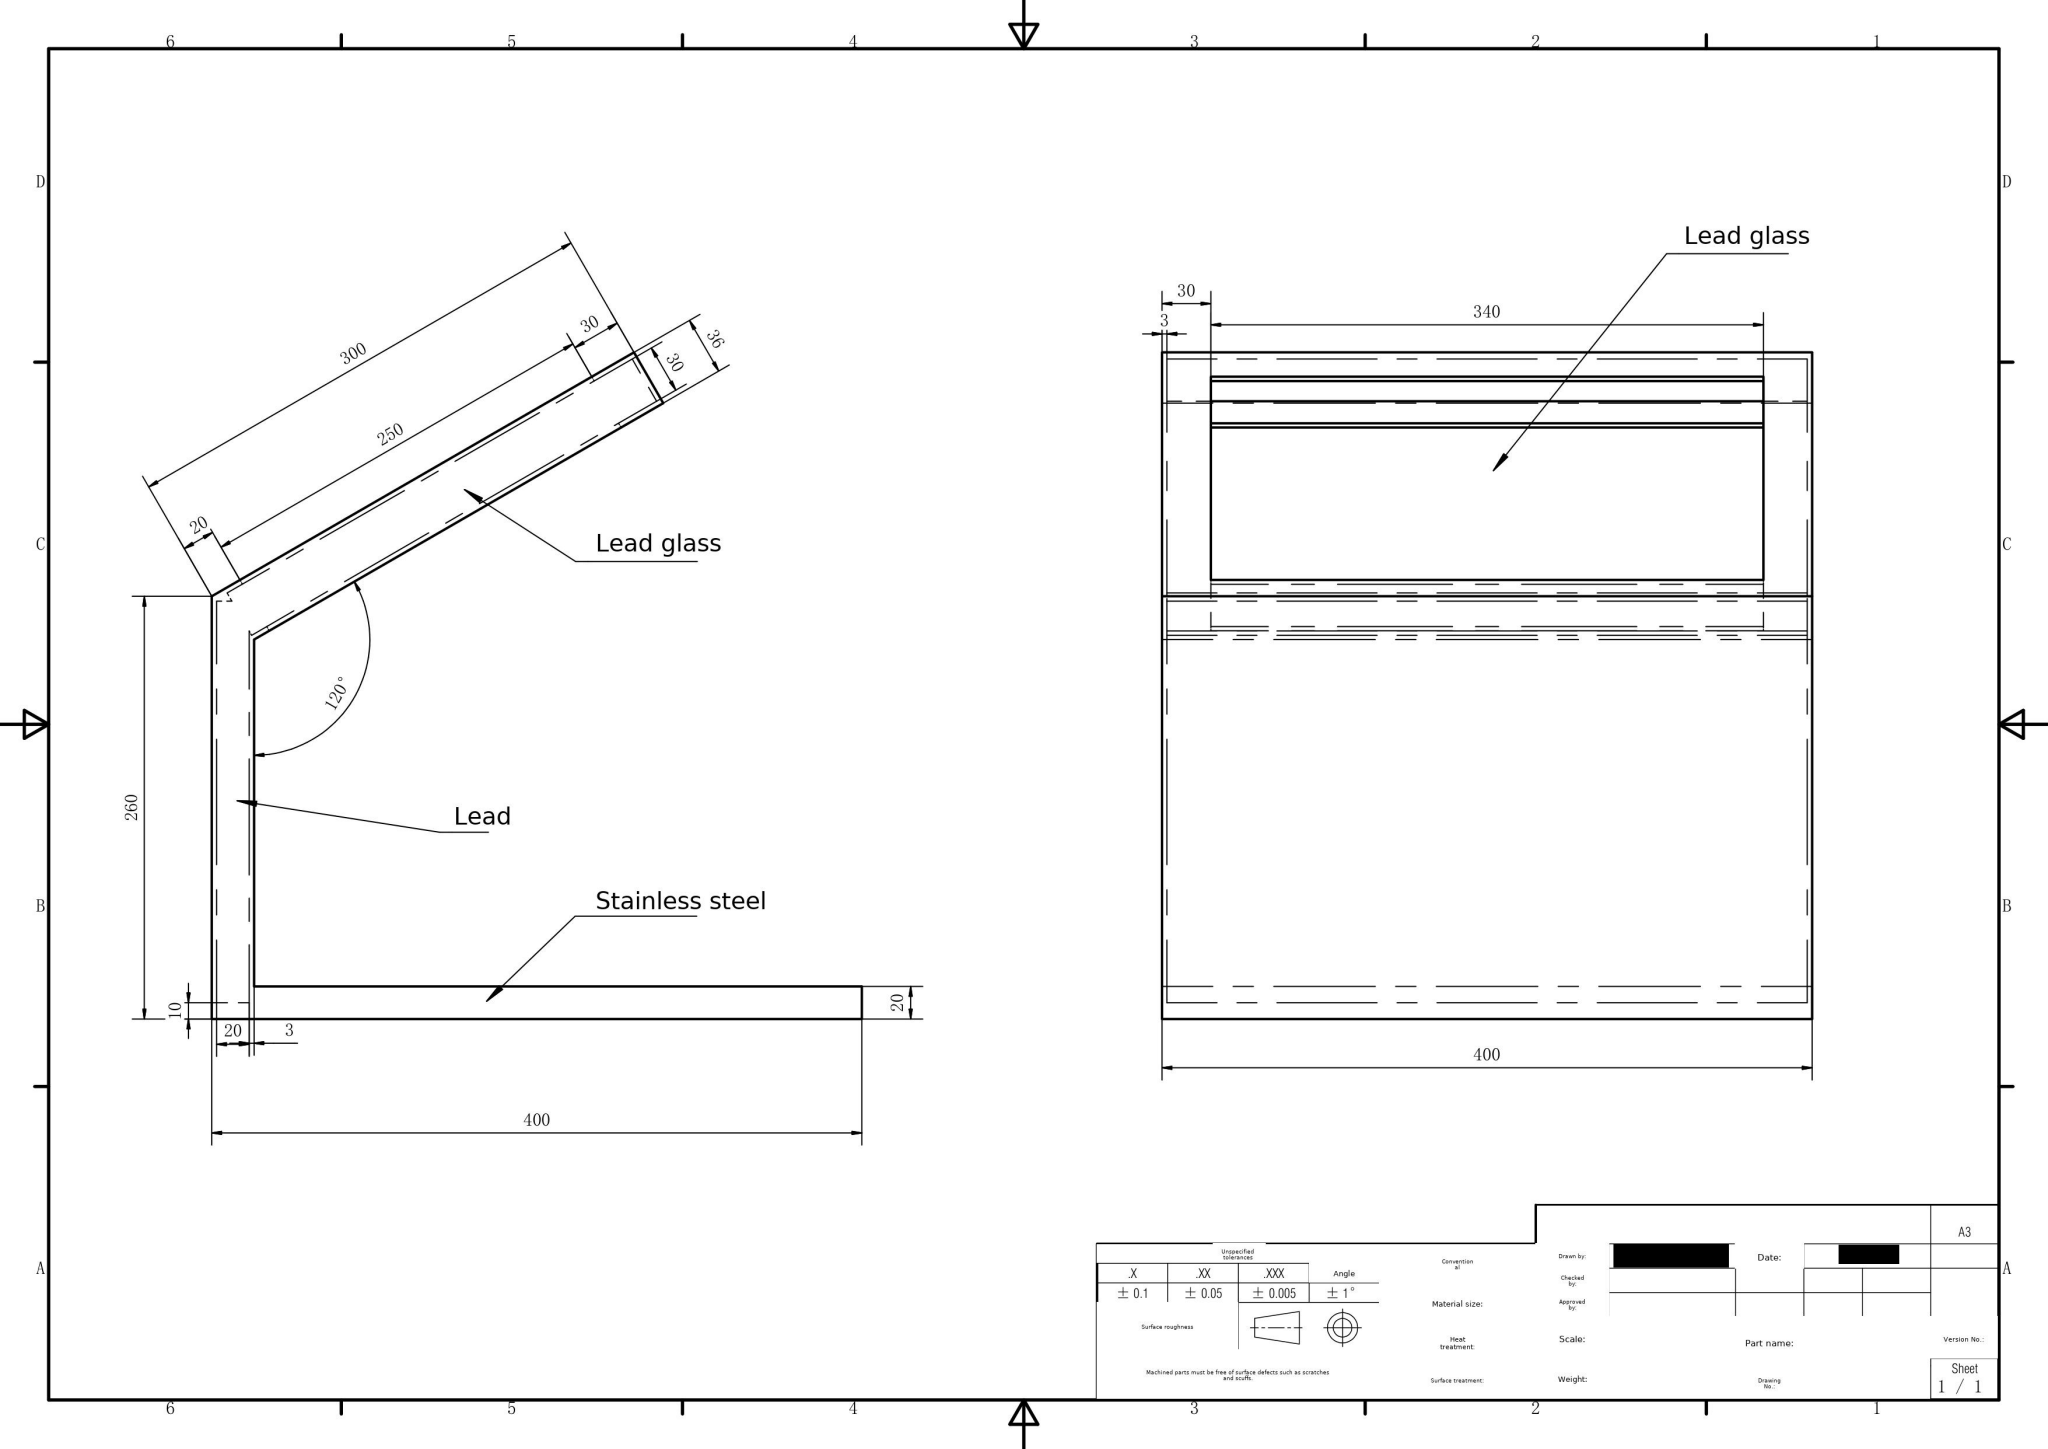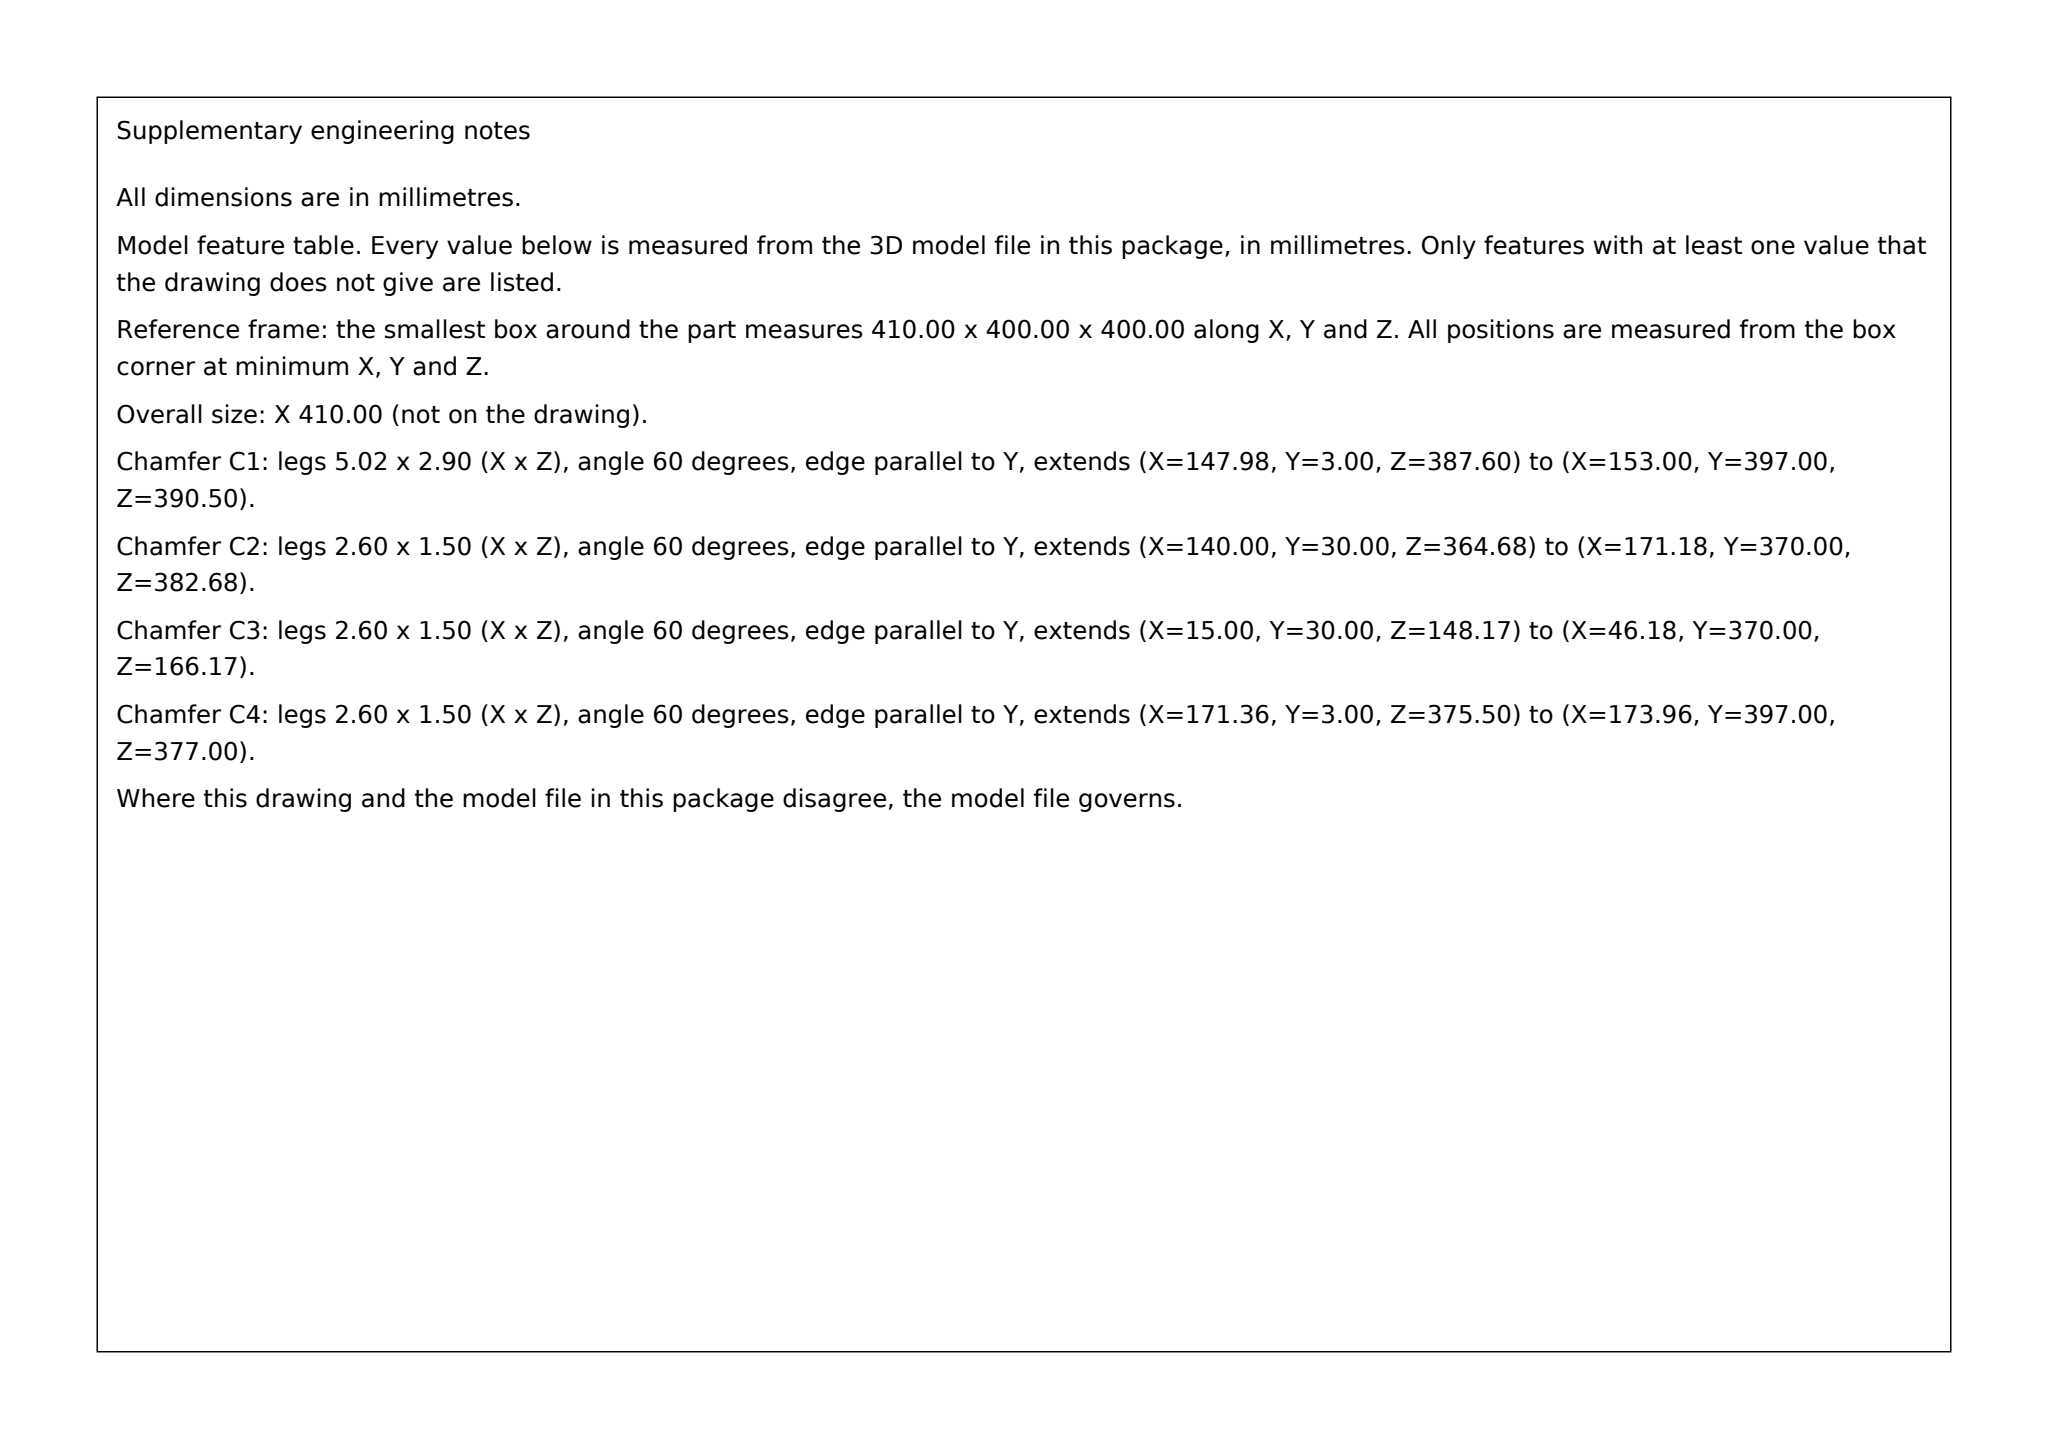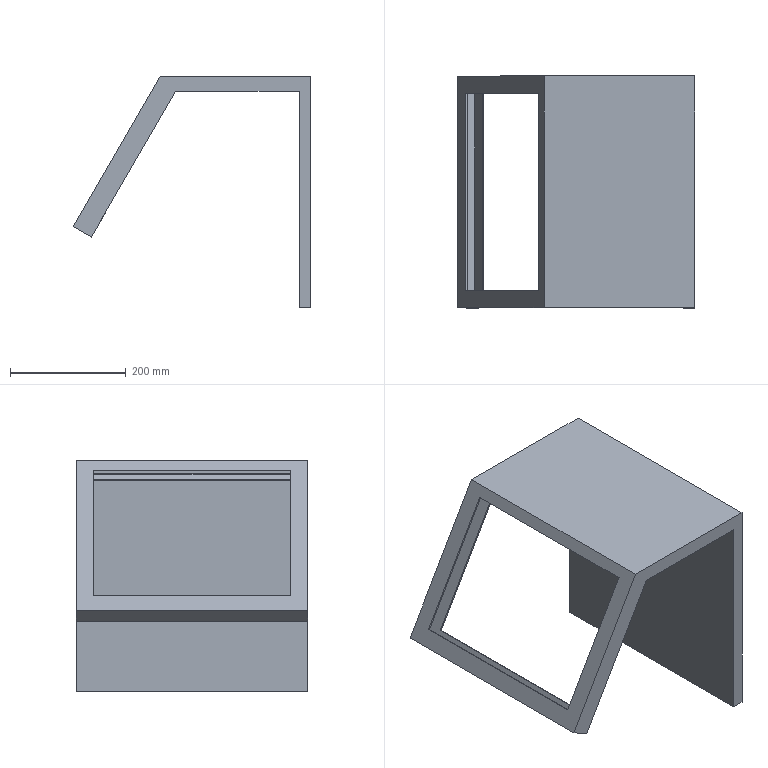Part | SolidWorks | mm | 1 solid | 29 faces | box 410 x 400 x 400 mm | volume 3992024 mm3 | plane 29
STEP:
#1=CARTESIAN_POINT('',(260.,400.,-400.));
#2=VERTEX_POINT('',#1);
#3=CARTESIAN_POINT('',(260.,400.,-0.));
#4=VERTEX_POINT('',#3);
#5=CARTESIAN_POINT('',(260.,400.,-0.));
#6=DIRECTION('',(0.,0.,1.));
#7=VECTOR('',#6,1000.);
#8=LINE('',#5,#7);
#9=EDGE_CURVE('',#2,#4,#8,.T.);
#10=ORIENTED_EDGE('',*,*,#9,.T.);
#11=CARTESIAN_POINT('',(260.,0.,-0.));
#12=VERTEX_POINT('',#11);
#13=CARTESIAN_POINT('',(260.,0.,-0.));
#14=DIRECTION('',(0.,-1.,0.));
#15=VECTOR('',#14,1000.);
#16=LINE('',#13,#15);
#17=EDGE_CURVE('',#4,#12,#16,.T.);
#18=ORIENTED_EDGE('',*,*,#17,.T.);
#19=CARTESIAN_POINT('',(260.,0.,-400.));
#20=VERTEX_POINT('',#19);
#21=CARTESIAN_POINT('',(260.,0.,-0.));
#22=DIRECTION('',(-0.,0.,-1.));
#23=VECTOR('',#22,1000.);
#24=LINE('',#21,#23);
#25=EDGE_CURVE('',#12,#20,#24,.T.);
#26=ORIENTED_EDGE('',*,*,#25,.T.);
#27=CARTESIAN_POINT('',(260.,0.,-400.));
#28=DIRECTION('',(0.,1.,0.));
#29=VECTOR('',#28,1000.);
#30=LINE('',#27,#29);
#31=EDGE_CURVE('',#20,#2,#30,.T.);
#32=ORIENTED_EDGE('',*,*,#31,.T.);
#33=EDGE_LOOP('',(#10,#18,#26,#32));
#34=FACE_OUTER_BOUND('',#33,.T.);
#35=CARTESIAN_POINT('',(260.,0.,-0.));
#36=DIRECTION('',(1.,0.,-0.));
#37=DIRECTION('',(-0.,0.,-1.));
#38=AXIS2_PLACEMENT_3D('',#35,#36,#37);
#39=PLANE('',#38);
#40=ADVANCED_FACE('',(#34),#39,.T.);
#41=CARTESIAN_POINT('',(0.,400.,0.));
#42=VERTEX_POINT('',#41);
#43=CARTESIAN_POINT('',(0.,400.,0.));
#44=DIRECTION('',(-1.,0.,0.));
#45=VECTOR('',#44,1000.);
#46=LINE('',#43,#45);
#47=EDGE_CURVE('',#4,#42,#46,.T.);
#48=ORIENTED_EDGE('',*,*,#47,.T.);
#49=CARTESIAN_POINT('',(0.,0.,-0.));
#50=VERTEX_POINT('',#49);
#51=CARTESIAN_POINT('',(0.,0.,0.));
#52=DIRECTION('',(0.,-1.,0.));
#53=VECTOR('',#52,1000.);
#54=LINE('',#51,#53);
#55=EDGE_CURVE('',#42,#50,#54,.T.);
#56=ORIENTED_EDGE('',*,*,#55,.T.);
#57=CARTESIAN_POINT('',(0.,0.,0.));
#58=DIRECTION('',(1.,0.,-0.));
#59=VECTOR('',#58,1000.);
#60=LINE('',#57,#59);
#61=EDGE_CURVE('',#50,#12,#60,.T.);
#62=ORIENTED_EDGE('',*,*,#61,.T.);
#63=ORIENTED_EDGE('',*,*,#17,.F.);
#64=EDGE_LOOP('',(#48,#56,#62,#63));
#65=FACE_OUTER_BOUND('',#64,.T.);
#66=CARTESIAN_POINT('',(0.,0.,0.));
#67=DIRECTION('',(0.,0.,1.));
#68=DIRECTION('',(1.,0.,-0.));
#69=AXIS2_PLACEMENT_3D('',#66,#67,#68);
#70=PLANE('',#69);
#71=ADVANCED_FACE('',(#65),#70,.T.);
#72=CARTESIAN_POINT('',(26.558,400.,-26.));
#73=VERTEX_POINT('',#72);
#74=CARTESIAN_POINT('',(-118.823,400.,-277.808));
#75=VERTEX_POINT('',#74);
#76=CARTESIAN_POINT('',(26.558,400.,-26.));
#77=DIRECTION('',(-0.5,0.,-0.866));
#78=VECTOR('',#77,1000.);
#79=LINE('',#76,#78);
#80=EDGE_CURVE('',#73,#75,#79,.T.);
#81=ORIENTED_EDGE('',*,*,#80,.T.);
#82=CARTESIAN_POINT('',(-150.,400.,-259.808));
#83=VERTEX_POINT('',#82);
#84=CARTESIAN_POINT('',(-118.823,400.,-277.808));
#85=DIRECTION('',(-0.866,0.,0.5));
#86=VECTOR('',#85,1000.);
#87=LINE('',#84,#86);
#88=EDGE_CURVE('',#75,#83,#87,.T.);
#89=ORIENTED_EDGE('',*,*,#88,.T.);
#90=CARTESIAN_POINT('',(-150.,400.,-259.808));
#91=DIRECTION('',(0.5,0.,0.866));
#92=VECTOR('',#91,1000.);
#93=LINE('',#90,#92);
#94=EDGE_CURVE('',#83,#42,#93,.T.);
#95=ORIENTED_EDGE('',*,*,#94,.T.);
#96=ORIENTED_EDGE('',*,*,#47,.F.);
#97=ORIENTED_EDGE('',*,*,#9,.F.);
#98=CARTESIAN_POINT('',(240.,400.,-400.));
#99=VERTEX_POINT('',#98);
#100=CARTESIAN_POINT('',(55.,400.,-400.));
#101=DIRECTION('',(-1.,0.,0.));
#102=VECTOR('',#101,1000.);
#103=LINE('',#100,#102);
#104=EDGE_CURVE('',#2,#99,#103,.T.);
#105=ORIENTED_EDGE('',*,*,#104,.T.);
#106=CARTESIAN_POINT('',(240.,400.,-26.));
#107=VERTEX_POINT('',#106);
#108=CARTESIAN_POINT('',(240.,400.,-200.));
#109=DIRECTION('',(0.,0.,1.));
#110=VECTOR('',#109,1000.);
#111=LINE('',#108,#110);
#112=EDGE_CURVE('',#99,#107,#111,.T.);
#113=ORIENTED_EDGE('',*,*,#112,.T.);
#114=CARTESIAN_POINT('',(55.,400.,-26.));
#115=DIRECTION('',(-1.,0.,0.));
#116=VECTOR('',#115,1000.);
#117=LINE('',#114,#116);
#118=EDGE_CURVE('',#107,#73,#117,.T.);
#119=ORIENTED_EDGE('',*,*,#118,.T.);
#120=EDGE_LOOP('',(#81,#89,#95,#96,#97,#105,#113,#119));
#121=FACE_OUTER_BOUND('',#120,.T.);
#122=CARTESIAN_POINT('',(55.,400.,-200.));
#123=DIRECTION('',(0.,1.,0.));
#124=DIRECTION('',(0.,0.,1.));
#125=AXIS2_PLACEMENT_3D('',#122,#123,#124);
#126=PLANE('',#125);
#127=ADVANCED_FACE('',(#121),#126,.T.);
#128=ORIENTED_EDGE('',*,*,#104,.F.);
#129=ORIENTED_EDGE('',*,*,#31,.F.);
#130=CARTESIAN_POINT('',(240.,0.,-400.));
#131=VERTEX_POINT('',#130);
#132=CARTESIAN_POINT('',(260.,0.,-400.));
#133=DIRECTION('',(-1.,0.,0.));
#134=VECTOR('',#133,1000.);
#135=LINE('',#132,#134);
#136=EDGE_CURVE('',#20,#131,#135,.T.);
#137=ORIENTED_EDGE('',*,*,#136,.T.);
#138=CARTESIAN_POINT('',(240.,0.,-400.));
#139=DIRECTION('',(0.,1.,0.));
#140=VECTOR('',#139,1000.);
#141=LINE('',#138,#140);
#142=EDGE_CURVE('',#131,#99,#141,.T.);
#143=ORIENTED_EDGE('',*,*,#142,.T.);
#144=EDGE_LOOP('',(#128,#129,#137,#143));
#145=FACE_OUTER_BOUND('',#144,.T.);
#146=CARTESIAN_POINT('',(260.,0.,-400.));
#147=DIRECTION('',(0.,0.,-1.));
#148=DIRECTION('',(-1.,0.,0.));
#149=AXIS2_PLACEMENT_3D('',#146,#147,#148);
#150=PLANE('',#149);
#151=ADVANCED_FACE('',(#145),#150,.T.);
#152=CARTESIAN_POINT('',(-118.823,0.,-277.808));
#153=VERTEX_POINT('',#152);
#154=CARTESIAN_POINT('',(-150.,0.,-259.808));
#155=VERTEX_POINT('',#154);
#156=CARTESIAN_POINT('',(-118.823,0.,-277.808));
#157=DIRECTION('',(-0.866,0.,0.5));
#158=VECTOR('',#157,1000.);
#159=LINE('',#156,#158);
#160=EDGE_CURVE('',#153,#155,#159,.T.);
#161=ORIENTED_EDGE('',*,*,#160,.F.);
#162=CARTESIAN_POINT('',(26.558,0.,-26.));
#163=VERTEX_POINT('',#162);
#164=CARTESIAN_POINT('',(26.558,0.,-26.));
#165=DIRECTION('',(-0.5,0.,-0.866));
#166=VECTOR('',#165,1000.);
#167=LINE('',#164,#166);
#168=EDGE_CURVE('',#163,#153,#167,.T.);
#169=ORIENTED_EDGE('',*,*,#168,.F.);
#170=CARTESIAN_POINT('',(240.,0.,-26.));
#171=VERTEX_POINT('',#170);
#172=CARTESIAN_POINT('',(55.,0.,-26.));
#173=DIRECTION('',(-1.,0.,0.));
#174=VECTOR('',#173,1000.);
#175=LINE('',#172,#174);
#176=EDGE_CURVE('',#171,#163,#175,.T.);
#177=ORIENTED_EDGE('',*,*,#176,.F.);
#178=CARTESIAN_POINT('',(240.,0.,-200.));
#179=DIRECTION('',(0.,0.,1.));
#180=VECTOR('',#179,1000.);
#181=LINE('',#178,#180);
#182=EDGE_CURVE('',#131,#171,#181,.T.);
#183=ORIENTED_EDGE('',*,*,#182,.F.);
#184=ORIENTED_EDGE('',*,*,#136,.F.);
#185=ORIENTED_EDGE('',*,*,#25,.F.);
#186=ORIENTED_EDGE('',*,*,#61,.F.);
#187=CARTESIAN_POINT('',(-150.,0.,-259.808));
#188=DIRECTION('',(0.5,0.,0.866));
#189=VECTOR('',#188,1000.);
#190=LINE('',#187,#189);
#191=EDGE_CURVE('',#155,#50,#190,.T.);
#192=ORIENTED_EDGE('',*,*,#191,.F.);
#193=EDGE_LOOP('',(#161,#169,#177,#183,#184,#185,#186,#192));
#194=FACE_OUTER_BOUND('',#193,.T.);
#195=CARTESIAN_POINT('',(55.,0.,-200.));
#196=DIRECTION('',(0.,1.,0.));
#197=DIRECTION('',(0.,0.,1.));
#198=AXIS2_PLACEMENT_3D('',#195,#196,#197);
#199=PLANE('',#198);
#200=ADVANCED_FACE('',(#194),#199,.F.);
#201=CARTESIAN_POINT('',(-135.,370.,-233.827));
#202=VERTEX_POINT('',#201);
#203=CARTESIAN_POINT('',(-10.,370.,-17.321));
#204=VERTEX_POINT('',#203);
#205=CARTESIAN_POINT('',(-150.,370.,-259.808));
#206=DIRECTION('',(0.5,0.,0.866));
#207=VECTOR('',#206,1000.);
#208=LINE('',#205,#207);
#209=EDGE_CURVE('',#202,#204,#208,.T.);
#210=ORIENTED_EDGE('',*,*,#209,.T.);
#211=CARTESIAN_POINT('',(-10.,30.,-17.321));
#212=VERTEX_POINT('',#211);
#213=CARTESIAN_POINT('',(-10.,0.,-17.321));
#214=DIRECTION('',(0.,-1.,0.));
#215=VECTOR('',#214,1000.);
#216=LINE('',#213,#215);
#217=EDGE_CURVE('',#204,#212,#216,.T.);
#218=ORIENTED_EDGE('',*,*,#217,.T.);
#219=CARTESIAN_POINT('',(-135.,30.,-233.827));
#220=VERTEX_POINT('',#219);
#221=CARTESIAN_POINT('',(-150.,30.,-259.808));
#222=DIRECTION('',(-0.5,0.,-0.866));
#223=VECTOR('',#222,1000.);
#224=LINE('',#221,#223);
#225=EDGE_CURVE('',#212,#220,#224,.T.);
#226=ORIENTED_EDGE('',*,*,#225,.T.);
#227=CARTESIAN_POINT('',(-135.,0.,-233.827));
#228=DIRECTION('',(0.,1.,0.));
#229=VECTOR('',#228,1000.);
#230=LINE('',#227,#229);
#231=EDGE_CURVE('',#220,#202,#230,.T.);
#232=ORIENTED_EDGE('',*,*,#231,.T.);
#233=EDGE_LOOP('',(#210,#218,#226,#232));
#234=FACE_BOUND('',#233,.T.);
#235=ORIENTED_EDGE('',*,*,#94,.F.);
#236=CARTESIAN_POINT('',(-150.,0.,-259.808));
#237=DIRECTION('',(0.,-1.,0.));
#238=VECTOR('',#237,1000.);
#239=LINE('',#236,#238);
#240=EDGE_CURVE('',#83,#155,#239,.T.);
#241=ORIENTED_EDGE('',*,*,#240,.T.);
#242=ORIENTED_EDGE('',*,*,#191,.T.);
#243=ORIENTED_EDGE('',*,*,#55,.F.);
#244=EDGE_LOOP('',(#235,#241,#242,#243));
#245=FACE_OUTER_BOUND('',#244,.T.);
#246=CARTESIAN_POINT('',(-150.,0.,-259.808));
#247=DIRECTION('',(-0.866,0.,0.5));
#248=DIRECTION('',(0.5,0.,0.866));
#249=AXIS2_PLACEMENT_3D('',#246,#247,#248);
#250=PLANE('',#249);
#251=ADVANCED_FACE('',(#234,#245),#250,.T.);
#252=ORIENTED_EDGE('',*,*,#88,.F.);
#253=CARTESIAN_POINT('',(-118.823,0.,-277.808));
#254=DIRECTION('',(0.,-1.,0.));
#255=VECTOR('',#254,1000.);
#256=LINE('',#253,#255);
#257=EDGE_CURVE('',#75,#153,#256,.T.);
#258=ORIENTED_EDGE('',*,*,#257,.T.);
#259=ORIENTED_EDGE('',*,*,#160,.T.);
#260=ORIENTED_EDGE('',*,*,#240,.F.);
#261=EDGE_LOOP('',(#252,#258,#259,#260));
#262=FACE_OUTER_BOUND('',#261,.T.);
#263=CARTESIAN_POINT('',(-118.823,0.,-277.808));
#264=DIRECTION('',(-0.5,0.,-0.866));
#265=DIRECTION('',(-0.866,0.,0.5));
#266=AXIS2_PLACEMENT_3D('',#263,#264,#265);
#267=PLANE('',#266);
#268=ADVANCED_FACE('',(#262),#267,.T.);
#269=CARTESIAN_POINT('',(21.177,370.,-35.321));
#270=VERTEX_POINT('',#269);
#271=CARTESIAN_POINT('',(-103.823,370.,-251.827));
#272=VERTEX_POINT('',#271);
#273=CARTESIAN_POINT('',(26.558,370.,-26.));
#274=DIRECTION('',(-0.5,0.,-0.866));
#275=VECTOR('',#274,1000.);
#276=LINE('',#273,#275);
#277=EDGE_CURVE('',#270,#272,#276,.T.);
#278=ORIENTED_EDGE('',*,*,#277,.T.);
#279=CARTESIAN_POINT('',(-103.823,30.,-251.827));
#280=VERTEX_POINT('',#279);
#281=CARTESIAN_POINT('',(-103.823,0.,-251.827));
#282=DIRECTION('',(0.,-1.,0.));
#283=VECTOR('',#282,1000.);
#284=LINE('',#281,#283);
#285=EDGE_CURVE('',#272,#280,#284,.T.);
#286=ORIENTED_EDGE('',*,*,#285,.T.);
#287=CARTESIAN_POINT('',(21.177,30.,-35.321));
#288=VERTEX_POINT('',#287);
#289=CARTESIAN_POINT('',(26.558,30.,-26.));
#290=DIRECTION('',(0.5,0.,0.866));
#291=VECTOR('',#290,1000.);
#292=LINE('',#289,#291);
#293=EDGE_CURVE('',#280,#288,#292,.T.);
#294=ORIENTED_EDGE('',*,*,#293,.T.);
#295=CARTESIAN_POINT('',(21.177,0.,-35.321));
#296=DIRECTION('',(0.,1.,0.));
#297=VECTOR('',#296,1000.);
#298=LINE('',#295,#297);
#299=EDGE_CURVE('',#288,#270,#298,.T.);
#300=ORIENTED_EDGE('',*,*,#299,.T.);
#301=EDGE_LOOP('',(#278,#286,#294,#300));
#302=FACE_BOUND('',#301,.T.);
#303=ORIENTED_EDGE('',*,*,#80,.F.);
#304=CARTESIAN_POINT('',(26.558,0.,-26.));
#305=DIRECTION('',(0.,-1.,0.));
#306=VECTOR('',#305,1000.);
#307=LINE('',#304,#306);
#308=EDGE_CURVE('',#73,#163,#307,.T.);
#309=ORIENTED_EDGE('',*,*,#308,.T.);
#310=ORIENTED_EDGE('',*,*,#168,.T.);
#311=ORIENTED_EDGE('',*,*,#257,.F.);
#312=EDGE_LOOP('',(#303,#309,#310,#311));
#313=FACE_OUTER_BOUND('',#312,.T.);
#314=CARTESIAN_POINT('',(26.558,0.,-26.));
#315=DIRECTION('',(0.866,0.,-0.5));
#316=DIRECTION('',(-0.5,0.,-0.866));
#317=AXIS2_PLACEMENT_3D('',#314,#315,#316);
#318=PLANE('',#317);
#319=ADVANCED_FACE('',(#302,#313),#318,.T.);
#320=ORIENTED_EDGE('',*,*,#118,.F.);
#321=CARTESIAN_POINT('',(240.,0.,-26.));
#322=DIRECTION('',(0.,-1.,0.));
#323=VECTOR('',#322,1000.);
#324=LINE('',#321,#323);
#325=EDGE_CURVE('',#107,#171,#324,.T.);
#326=ORIENTED_EDGE('',*,*,#325,.T.);
#327=ORIENTED_EDGE('',*,*,#176,.T.);
#328=ORIENTED_EDGE('',*,*,#308,.F.);
#329=EDGE_LOOP('',(#320,#326,#327,#328));
#330=FACE_OUTER_BOUND('',#329,.T.);
#331=CARTESIAN_POINT('',(240.,0.,-26.));
#332=DIRECTION('',(-0.,0.,-1.));
#333=DIRECTION('',(-1.,0.,0.));
#334=AXIS2_PLACEMENT_3D('',#331,#332,#333);
#335=PLANE('',#334);
#336=ADVANCED_FACE('',(#330),#335,.T.);
#337=ORIENTED_EDGE('',*,*,#112,.F.);
#338=ORIENTED_EDGE('',*,*,#142,.F.);
#339=ORIENTED_EDGE('',*,*,#182,.T.);
#340=ORIENTED_EDGE('',*,*,#325,.F.);
#341=EDGE_LOOP('',(#337,#338,#339,#340));
#342=FACE_OUTER_BOUND('',#341,.T.);
#343=CARTESIAN_POINT('',(240.,0.,-400.));
#344=DIRECTION('',(-1.,0.,0.));
#345=DIRECTION('',(0.,0.,1.));
#346=AXIS2_PLACEMENT_3D('',#343,#344,#345);
#347=PLANE('',#346);
#348=ADVANCED_FACE('',(#342),#347,.T.);
#349=CARTESIAN_POINT('',(-7.402,30.,-18.821));
#350=VERTEX_POINT('',#349);
#351=CARTESIAN_POINT('',(-10.,30.,-17.321));
#352=DIRECTION('',(0.866,0.,-0.5));
#353=VECTOR('',#352,1000.);
#354=LINE('',#351,#353);
#355=EDGE_CURVE('',#212,#350,#354,.T.);
#356=ORIENTED_EDGE('',*,*,#355,.F.);
#357=ORIENTED_EDGE('',*,*,#217,.F.);
#358=CARTESIAN_POINT('',(-7.402,370.,-18.821));
#359=VERTEX_POINT('',#358);
#360=CARTESIAN_POINT('',(-10.,370.,-17.321));
#361=DIRECTION('',(-0.866,0.,0.5));
#362=VECTOR('',#361,1000.);
#363=LINE('',#360,#362);
#364=EDGE_CURVE('',#359,#204,#363,.T.);
#365=ORIENTED_EDGE('',*,*,#364,.F.);
#366=CARTESIAN_POINT('',(-7.402,370.,-18.821));
#367=DIRECTION('',(-0.,1.,-0.));
#368=VECTOR('',#367,1000.);
#369=LINE('',#366,#368);
#370=EDGE_CURVE('',#350,#359,#369,.T.);
#371=ORIENTED_EDGE('',*,*,#370,.F.);
#372=EDGE_LOOP('',(#356,#357,#365,#371));
#373=FACE_OUTER_BOUND('',#372,.T.);
#374=CARTESIAN_POINT('',(-10.,370.,-17.321));
#375=DIRECTION('',(0.5,0.,0.866));
#376=DIRECTION('',(0.866,0.,-0.5));
#377=AXIS2_PLACEMENT_3D('',#374,#375,#376);
#378=PLANE('',#377);
#379=ADVANCED_FACE('',(#373),#378,.F.);
#380=ORIENTED_EDGE('',*,*,#364,.T.);
#381=ORIENTED_EDGE('',*,*,#209,.F.);
#382=CARTESIAN_POINT('',(-132.402,370.,-235.327));
#383=VERTEX_POINT('',#382);
#384=CARTESIAN_POINT('',(-132.402,370.,-235.327));
#385=DIRECTION('',(-0.866,0.,0.5));
#386=VECTOR('',#385,1000.);
#387=LINE('',#384,#386);
#388=EDGE_CURVE('',#383,#202,#387,.T.);
#389=ORIENTED_EDGE('',*,*,#388,.F.);
#390=CARTESIAN_POINT('',(-7.402,370.,-18.821));
#391=DIRECTION('',(-0.5,0.,-0.866));
#392=VECTOR('',#391,1000.);
#393=LINE('',#390,#392);
#394=EDGE_CURVE('',#359,#383,#393,.T.);
#395=ORIENTED_EDGE('',*,*,#394,.F.);
#396=EDGE_LOOP('',(#380,#381,#389,#395));
#397=FACE_OUTER_BOUND('',#396,.T.);
#398=CARTESIAN_POINT('',(-135.,370.,-233.827));
#399=DIRECTION('',(0.,1.,0.));
#400=DIRECTION('',(0.,0.,1.));
#401=AXIS2_PLACEMENT_3D('',#398,#399,#400);
#402=PLANE('',#401);
#403=ADVANCED_FACE('',(#397),#402,.F.);
#404=ORIENTED_EDGE('',*,*,#388,.T.);
#405=ORIENTED_EDGE('',*,*,#231,.F.);
#406=CARTESIAN_POINT('',(-132.402,30.,-235.327));
#407=VERTEX_POINT('',#406);
#408=CARTESIAN_POINT('',(-135.,30.,-233.827));
#409=DIRECTION('',(-0.866,0.,0.5));
#410=VECTOR('',#409,1000.);
#411=LINE('',#408,#410);
#412=EDGE_CURVE('',#407,#220,#411,.T.);
#413=ORIENTED_EDGE('',*,*,#412,.F.);
#414=CARTESIAN_POINT('',(-132.402,30.,-235.327));
#415=DIRECTION('',(0.,-1.,0.));
#416=VECTOR('',#415,1000.);
#417=LINE('',#414,#416);
#418=EDGE_CURVE('',#383,#407,#417,.T.);
#419=ORIENTED_EDGE('',*,*,#418,.F.);
#420=EDGE_LOOP('',(#404,#405,#413,#419));
#421=FACE_OUTER_BOUND('',#420,.T.);
#422=CARTESIAN_POINT('',(-135.,30.,-233.827));
#423=DIRECTION('',(-0.5,-0.,-0.866));
#424=DIRECTION('',(-0.866,0.,0.5));
#425=AXIS2_PLACEMENT_3D('',#422,#423,#424);
#426=PLANE('',#425);
#427=ADVANCED_FACE('',(#421),#426,.F.);
#428=ORIENTED_EDGE('',*,*,#412,.T.);
#429=ORIENTED_EDGE('',*,*,#225,.F.);
#430=ORIENTED_EDGE('',*,*,#355,.T.);
#431=CARTESIAN_POINT('',(-132.402,30.,-235.327));
#432=DIRECTION('',(0.5,0.,0.866));
#433=VECTOR('',#432,1000.);
#434=LINE('',#431,#433);
#435=EDGE_CURVE('',#407,#350,#434,.T.);
#436=ORIENTED_EDGE('',*,*,#435,.F.);
#437=EDGE_LOOP('',(#428,#429,#430,#436));
#438=FACE_OUTER_BOUND('',#437,.T.);
#439=CARTESIAN_POINT('',(-10.,30.,-17.321));
#440=DIRECTION('',(0.,-1.,0.));
#441=DIRECTION('',(0.,0.,-1.));
#442=AXIS2_PLACEMENT_3D('',#439,#440,#441);
#443=PLANE('',#442);
#444=ADVANCED_FACE('',(#438),#443,.F.);
#445=CARTESIAN_POINT('',(-106.421,30.,-250.327));
#446=VERTEX_POINT('',#445);
#447=CARTESIAN_POINT('',(-135.,30.,-233.827));
#448=DIRECTION('',(-0.866,0.,0.5));
#449=VECTOR('',#448,1000.);
#450=LINE('',#447,#449);
#451=EDGE_CURVE('',#280,#446,#450,.T.);
#452=ORIENTED_EDGE('',*,*,#451,.F.);
#453=ORIENTED_EDGE('',*,*,#285,.F.);
#454=CARTESIAN_POINT('',(-106.421,370.,-250.327));
#455=VERTEX_POINT('',#454);
#456=CARTESIAN_POINT('',(-135.,370.,-233.827));
#457=DIRECTION('',(0.866,0.,-0.5));
#458=VECTOR('',#457,1000.);
#459=LINE('',#456,#458);
#460=EDGE_CURVE('',#455,#272,#459,.T.);
#461=ORIENTED_EDGE('',*,*,#460,.F.);
#462=CARTESIAN_POINT('',(-106.421,30.,-250.327));
#463=DIRECTION('',(-0.,1.,-0.));
#464=VECTOR('',#463,1000.);
#465=LINE('',#462,#464);
#466=EDGE_CURVE('',#446,#455,#465,.T.);
#467=ORIENTED_EDGE('',*,*,#466,.F.);
#468=EDGE_LOOP('',(#452,#453,#461,#467));
#469=FACE_OUTER_BOUND('',#468,.T.);
#470=CARTESIAN_POINT('',(-135.,30.,-233.827));
#471=DIRECTION('',(-0.5,-0.,-0.866));
#472=DIRECTION('',(-0.866,0.,0.5));
#473=AXIS2_PLACEMENT_3D('',#470,#471,#472);
#474=PLANE('',#473);
#475=ADVANCED_FACE('',(#469),#474,.F.);
#476=ORIENTED_EDGE('',*,*,#460,.T.);
#477=ORIENTED_EDGE('',*,*,#277,.F.);
#478=CARTESIAN_POINT('',(18.579,370.,-33.821));
#479=VERTEX_POINT('',#478);
#480=CARTESIAN_POINT('',(18.579,370.,-33.821));
#481=DIRECTION('',(0.866,0.,-0.5));
#482=VECTOR('',#481,1000.);
#483=LINE('',#480,#482);
#484=EDGE_CURVE('',#479,#270,#483,.T.);
#485=ORIENTED_EDGE('',*,*,#484,.F.);
#486=CARTESIAN_POINT('',(-106.421,370.,-250.327));
#487=DIRECTION('',(0.5,0.,0.866));
#488=VECTOR('',#487,1000.);
#489=LINE('',#486,#488);
#490=EDGE_CURVE('',#455,#479,#489,.T.);
#491=ORIENTED_EDGE('',*,*,#490,.F.);
#492=EDGE_LOOP('',(#476,#477,#485,#491));
#493=FACE_OUTER_BOUND('',#492,.T.);
#494=CARTESIAN_POINT('',(-135.,370.,-233.827));
#495=DIRECTION('',(0.,1.,0.));
#496=DIRECTION('',(0.,0.,1.));
#497=AXIS2_PLACEMENT_3D('',#494,#495,#496);
#498=PLANE('',#497);
#499=ADVANCED_FACE('',(#493),#498,.F.);
#500=ORIENTED_EDGE('',*,*,#484,.T.);
#501=ORIENTED_EDGE('',*,*,#299,.F.);
#502=CARTESIAN_POINT('',(18.579,30.,-33.821));
#503=VERTEX_POINT('',#502);
#504=CARTESIAN_POINT('',(-10.,30.,-17.321));
#505=DIRECTION('',(0.866,0.,-0.5));
#506=VECTOR('',#505,1000.);
#507=LINE('',#504,#506);
#508=EDGE_CURVE('',#503,#288,#507,.T.);
#509=ORIENTED_EDGE('',*,*,#508,.F.);
#510=CARTESIAN_POINT('',(18.579,370.,-33.821));
#511=DIRECTION('',(0.,-1.,0.));
#512=VECTOR('',#511,1000.);
#513=LINE('',#510,#512);
#514=EDGE_CURVE('',#479,#503,#513,.T.);
#515=ORIENTED_EDGE('',*,*,#514,.F.);
#516=EDGE_LOOP('',(#500,#501,#509,#515));
#517=FACE_OUTER_BOUND('',#516,.T.);
#518=CARTESIAN_POINT('',(-10.,370.,-17.321));
#519=DIRECTION('',(0.5,0.,0.866));
#520=DIRECTION('',(0.866,0.,-0.5));
#521=AXIS2_PLACEMENT_3D('',#518,#519,#520);
#522=PLANE('',#521);
#523=ADVANCED_FACE('',(#517),#522,.F.);
#524=ORIENTED_EDGE('',*,*,#508,.T.);
#525=ORIENTED_EDGE('',*,*,#293,.F.);
#526=ORIENTED_EDGE('',*,*,#451,.T.);
#527=CARTESIAN_POINT('',(18.579,30.,-33.821));
#528=DIRECTION('',(-0.5,0.,-0.866));
#529=VECTOR('',#528,1000.);
#530=LINE('',#527,#529);
#531=EDGE_CURVE('',#503,#446,#530,.T.);
#532=ORIENTED_EDGE('',*,*,#531,.F.);
#533=EDGE_LOOP('',(#524,#525,#526,#532));
#534=FACE_OUTER_BOUND('',#533,.T.);
#535=CARTESIAN_POINT('',(-10.,30.,-17.321));
#536=DIRECTION('',(0.,-1.,0.));
#537=DIRECTION('',(0.,0.,-1.));
#538=AXIS2_PLACEMENT_3D('',#535,#536,#537);
#539=PLANE('',#538);
#540=ADVANCED_FACE('',(#534),#539,.F.);
#541=ORIENTED_EDGE('',*,*,#418,.T.);
#542=ORIENTED_EDGE('',*,*,#435,.T.);
#543=ORIENTED_EDGE('',*,*,#370,.T.);
#544=ORIENTED_EDGE('',*,*,#394,.T.);
#545=EDGE_LOOP('',(#541,#542,#543,#544));
#546=FACE_BOUND('',#545,.T.);
#547=CARTESIAN_POINT('',(-145.902,3.,-258.71));
#548=VERTEX_POINT('',#547);
#549=CARTESIAN_POINT('',(-2.021,3.,-9.5));
#550=VERTEX_POINT('',#549);
#551=CARTESIAN_POINT('',(-73.961,3.,-134.105));
#552=DIRECTION('',(0.5,0.,0.866));
#553=VECTOR('',#552,1000.);
#554=LINE('',#551,#553);
#555=EDGE_CURVE('',#548,#550,#554,.T.);
#556=ORIENTED_EDGE('',*,*,#555,.F.);
#557=CARTESIAN_POINT('',(-145.902,397.,-258.71));
#558=VERTEX_POINT('',#557);
#559=CARTESIAN_POINT('',(-145.902,200.,-258.71));
#560=DIRECTION('',(0.,-1.,0.));
#561=VECTOR('',#560,1000.);
#562=LINE('',#559,#561);
#563=EDGE_CURVE('',#558,#548,#562,.T.);
#564=ORIENTED_EDGE('',*,*,#563,.F.);
#565=CARTESIAN_POINT('',(-2.021,397.,-9.5));
#566=VERTEX_POINT('',#565);
#567=CARTESIAN_POINT('',(-73.961,397.,-134.105));
#568=DIRECTION('',(-0.5,0.,-0.866));
#569=VECTOR('',#568,1000.);
#570=LINE('',#567,#569);
#571=EDGE_CURVE('',#566,#558,#570,.T.);
#572=ORIENTED_EDGE('',*,*,#571,.F.);
#573=CARTESIAN_POINT('',(-2.021,200.,-9.5));
#574=DIRECTION('',(0.,1.,0.));
#575=VECTOR('',#574,1000.);
#576=LINE('',#573,#575);
#577=EDGE_CURVE('',#550,#566,#576,.T.);
#578=ORIENTED_EDGE('',*,*,#577,.F.);
#579=EDGE_LOOP('',(#556,#564,#572,#578));
#580=FACE_OUTER_BOUND('',#579,.T.);
#581=CARTESIAN_POINT('',(-73.961,200.,-134.105));
#582=DIRECTION('',(-0.866,0.,0.5));
#583=DIRECTION('',(0.5,0.,0.866));
#584=AXIS2_PLACEMENT_3D('',#581,#582,#583);
#585=PLANE('',#584);
#586=ADVANCED_FACE('',(#546,#580),#585,.F.);
#587=ORIENTED_EDGE('',*,*,#514,.T.);
#588=ORIENTED_EDGE('',*,*,#531,.T.);
#589=ORIENTED_EDGE('',*,*,#466,.T.);
#590=ORIENTED_EDGE('',*,*,#490,.T.);
#591=EDGE_LOOP('',(#587,#588,#589,#590));
#592=FACE_BOUND('',#591,.T.);
#593=CARTESIAN_POINT('',(-119.921,397.,-273.71));
#594=VERTEX_POINT('',#593);
#595=CARTESIAN_POINT('',(23.96,397.,-24.5));
#596=VERTEX_POINT('',#595);
#597=CARTESIAN_POINT('',(-47.981,397.,-149.105));
#598=DIRECTION('',(0.5,0.,0.866));
#599=VECTOR('',#598,1000.);
#600=LINE('',#597,#599);
#601=EDGE_CURVE('',#594,#596,#600,.T.);
#602=ORIENTED_EDGE('',*,*,#601,.F.);
#603=CARTESIAN_POINT('',(-119.921,3.,-273.71));
#604=VERTEX_POINT('',#603);
#605=CARTESIAN_POINT('',(-119.921,200.,-273.71));
#606=DIRECTION('',(0.,1.,0.));
#607=VECTOR('',#606,1000.);
#608=LINE('',#605,#607);
#609=EDGE_CURVE('',#604,#594,#608,.T.);
#610=ORIENTED_EDGE('',*,*,#609,.F.);
#611=CARTESIAN_POINT('',(23.96,3.,-24.5));
#612=VERTEX_POINT('',#611);
#613=CARTESIAN_POINT('',(-47.981,3.,-149.105));
#614=DIRECTION('',(-0.5,0.,-0.866));
#615=VECTOR('',#614,1000.);
#616=LINE('',#613,#615);
#617=EDGE_CURVE('',#612,#604,#616,.T.);
#618=ORIENTED_EDGE('',*,*,#617,.F.);
#619=CARTESIAN_POINT('',(23.96,200.,-24.5));
#620=DIRECTION('',(0.,-1.,0.));
#621=VECTOR('',#620,1000.);
#622=LINE('',#619,#621);
#623=EDGE_CURVE('',#596,#612,#622,.T.);
#624=ORIENTED_EDGE('',*,*,#623,.F.);
#625=EDGE_LOOP('',(#602,#610,#618,#624));
#626=FACE_OUTER_BOUND('',#625,.T.);
#627=CARTESIAN_POINT('',(-47.981,200.,-149.105));
#628=DIRECTION('',(0.866,0.,-0.5));
#629=DIRECTION('',(-0.5,0.,-0.866));
#630=AXIS2_PLACEMENT_3D('',#627,#628,#629);
#631=PLANE('',#630);
#632=ADVANCED_FACE('',(#592,#626),#631,.F.);
#633=CARTESIAN_POINT('',(3.,3.,-12.399));
#634=VERTEX_POINT('',#633);
#635=CARTESIAN_POINT('',(-2.021,3.,-9.5));
#636=DIRECTION('',(0.866,0.,-0.5));
#637=VECTOR('',#636,1000.);
#638=LINE('',#635,#637);
#639=EDGE_CURVE('',#550,#634,#638,.T.);
#640=ORIENTED_EDGE('',*,*,#639,.F.);
#641=ORIENTED_EDGE('',*,*,#577,.T.);
#642=CARTESIAN_POINT('',(3.,397.,-12.399));
#643=VERTEX_POINT('',#642);
#644=CARTESIAN_POINT('',(-2.021,397.,-9.5));
#645=DIRECTION('',(-0.866,0.,0.5));
#646=VECTOR('',#645,1000.);
#647=LINE('',#644,#646);
#648=EDGE_CURVE('',#643,#566,#647,.T.);
#649=ORIENTED_EDGE('',*,*,#648,.F.);
#650=CARTESIAN_POINT('',(3.,397.,-12.399));
#651=DIRECTION('',(-0.,1.,-0.));
#652=VECTOR('',#651,1000.);
#653=LINE('',#650,#652);
#654=EDGE_CURVE('',#634,#643,#653,.T.);
#655=ORIENTED_EDGE('',*,*,#654,.F.);
#656=EDGE_LOOP('',(#640,#641,#649,#655));
#657=FACE_OUTER_BOUND('',#656,.T.);
#658=CARTESIAN_POINT('',(-2.021,397.,-9.5));
#659=DIRECTION('',(0.5,0.,0.866));
#660=DIRECTION('',(0.866,0.,-0.5));
#661=AXIS2_PLACEMENT_3D('',#658,#659,#660);
#662=PLANE('',#661);
#663=ADVANCED_FACE('',(#657),#662,.F.);
#664=CARTESIAN_POINT('',(21.362,3.,-23.));
#665=VERTEX_POINT('',#664);
#666=CARTESIAN_POINT('',(250.,3.,-23.));
#667=VERTEX_POINT('',#666);
#668=CARTESIAN_POINT('',(-2.021,3.,-23.));
#669=DIRECTION('',(1.,0.,0.));
#670=VECTOR('',#669,1000.);
#671=LINE('',#668,#670);
#672=EDGE_CURVE('',#665,#667,#671,.T.);
#673=ORIENTED_EDGE('',*,*,#672,.F.);
#674=CARTESIAN_POINT('',(23.96,3.,-24.5));
#675=DIRECTION('',(-0.866,0.,0.5));
#676=VECTOR('',#675,1000.);
#677=LINE('',#674,#676);
#678=EDGE_CURVE('',#612,#665,#677,.T.);
#679=ORIENTED_EDGE('',*,*,#678,.F.);
#680=ORIENTED_EDGE('',*,*,#617,.T.);
#681=CARTESIAN_POINT('',(-145.902,3.,-258.71));
#682=DIRECTION('',(0.866,0.,-0.5));
#683=VECTOR('',#682,1000.);
#684=LINE('',#681,#683);
#685=EDGE_CURVE('',#548,#604,#684,.T.);
#686=ORIENTED_EDGE('',*,*,#685,.F.);
#687=ORIENTED_EDGE('',*,*,#555,.T.);
#688=ORIENTED_EDGE('',*,*,#639,.T.);
#689=CARTESIAN_POINT('',(3.,3.,-3.));
#690=VERTEX_POINT('',#689);
#691=CARTESIAN_POINT('',(3.,3.,-9.5));
#692=DIRECTION('',(0.,0.,-1.));
#693=VECTOR('',#692,1000.);
#694=LINE('',#691,#693);
#695=EDGE_CURVE('',#690,#634,#694,.T.);
#696=ORIENTED_EDGE('',*,*,#695,.F.);
#697=CARTESIAN_POINT('',(250.,3.,-3.));
#698=VERTEX_POINT('',#697);
#699=CARTESIAN_POINT('',(-2.021,3.,-3.));
#700=DIRECTION('',(-1.,0.,0.));
#701=VECTOR('',#700,1000.);
#702=LINE('',#699,#701);
#703=EDGE_CURVE('',#698,#690,#702,.T.);
#704=ORIENTED_EDGE('',*,*,#703,.F.);
#705=CARTESIAN_POINT('',(250.,3.,-9.5));
#706=DIRECTION('',(0.,0.,1.));
#707=VECTOR('',#706,1000.);
#708=LINE('',#705,#707);
#709=EDGE_CURVE('',#667,#698,#708,.T.);
#710=ORIENTED_EDGE('',*,*,#709,.F.);
#711=EDGE_LOOP('',(#673,#679,#680,#686,#687,#688,#696,#704,#710));
#712=FACE_OUTER_BOUND('',#711,.T.);
#713=CARTESIAN_POINT('',(-2.021,3.,-9.5));
#714=DIRECTION('',(0.,-1.,0.));
#715=DIRECTION('',(0.,0.,-1.));
#716=AXIS2_PLACEMENT_3D('',#713,#714,#715);
#717=PLANE('',#716);
#718=ADVANCED_FACE('',(#712),#717,.F.);
#719=ORIENTED_EDGE('',*,*,#685,.T.);
#720=ORIENTED_EDGE('',*,*,#609,.T.);
#721=CARTESIAN_POINT('',(-145.902,397.,-258.71));
#722=DIRECTION('',(0.866,0.,-0.5));
#723=VECTOR('',#722,1000.);
#724=LINE('',#721,#723);
#725=EDGE_CURVE('',#558,#594,#724,.T.);
#726=ORIENTED_EDGE('',*,*,#725,.F.);
#727=ORIENTED_EDGE('',*,*,#563,.T.);
#728=EDGE_LOOP('',(#719,#720,#726,#727));
#729=FACE_OUTER_BOUND('',#728,.T.);
#730=CARTESIAN_POINT('',(-145.902,3.,-258.71));
#731=DIRECTION('',(-0.5,-0.,-0.866));
#732=DIRECTION('',(-0.866,0.,0.5));
#733=AXIS2_PLACEMENT_3D('',#730,#731,#732);
#734=PLANE('',#733);
#735=ADVANCED_FACE('',(#729),#734,.F.);
#736=CARTESIAN_POINT('',(3.,397.,-3.));
#737=VERTEX_POINT('',#736);
#738=CARTESIAN_POINT('',(250.,397.,-3.));
#739=VERTEX_POINT('',#738);
#740=CARTESIAN_POINT('',(-145.902,397.,-3.));
#741=DIRECTION('',(1.,0.,0.));
#742=VECTOR('',#741,1000.);
#743=LINE('',#740,#742);
#744=EDGE_CURVE('',#737,#739,#743,.T.);
#745=ORIENTED_EDGE('',*,*,#744,.F.);
#746=CARTESIAN_POINT('',(3.,397.,-258.71));
#747=DIRECTION('',(0.,0.,1.));
#748=VECTOR('',#747,1000.);
#749=LINE('',#746,#748);
#750=EDGE_CURVE('',#643,#737,#749,.T.);
#751=ORIENTED_EDGE('',*,*,#750,.F.);
#752=ORIENTED_EDGE('',*,*,#648,.T.);
#753=ORIENTED_EDGE('',*,*,#571,.T.);
#754=ORIENTED_EDGE('',*,*,#725,.T.);
#755=ORIENTED_EDGE('',*,*,#601,.T.);
#756=CARTESIAN_POINT('',(21.362,397.,-23.));
#757=VERTEX_POINT('',#756);
#758=CARTESIAN_POINT('',(21.362,397.,-23.));
#759=DIRECTION('',(0.866,0.,-0.5));
#760=VECTOR('',#759,1000.);
#761=LINE('',#758,#760);
#762=EDGE_CURVE('',#757,#596,#761,.T.);
#763=ORIENTED_EDGE('',*,*,#762,.F.);
#764=CARTESIAN_POINT('',(250.,397.,-23.));
#765=VERTEX_POINT('',#764);
#766=CARTESIAN_POINT('',(-145.902,397.,-23.));
#767=DIRECTION('',(-1.,0.,0.));
#768=VECTOR('',#767,1000.);
#769=LINE('',#766,#768);
#770=EDGE_CURVE('',#765,#757,#769,.T.);
#771=ORIENTED_EDGE('',*,*,#770,.F.);
#772=CARTESIAN_POINT('',(250.,397.,-258.71));
#773=DIRECTION('',(0.,0.,-1.));
#774=VECTOR('',#773,1000.);
#775=LINE('',#772,#774);
#776=EDGE_CURVE('',#739,#765,#775,.T.);
#777=ORIENTED_EDGE('',*,*,#776,.F.);
#778=EDGE_LOOP('',(#745,#751,#752,#753,#754,#755,#763,#771,#777));
#779=FACE_OUTER_BOUND('',#778,.T.);
#780=CARTESIAN_POINT('',(-145.902,397.,-258.71));
#781=DIRECTION('',(0.,1.,0.));
#782=DIRECTION('',(0.,0.,1.));
#783=AXIS2_PLACEMENT_3D('',#780,#781,#782);
#784=PLANE('',#783);
#785=ADVANCED_FACE('',(#779),#784,.F.);
#786=ORIENTED_EDGE('',*,*,#762,.T.);
#787=ORIENTED_EDGE('',*,*,#623,.T.);
#788=ORIENTED_EDGE('',*,*,#678,.T.);
#789=CARTESIAN_POINT('',(21.362,397.,-23.));
#790=DIRECTION('',(0.,-1.,0.));
#791=VECTOR('',#790,1000.);
#792=LINE('',#789,#791);
#793=EDGE_CURVE('',#757,#665,#792,.T.);
#794=ORIENTED_EDGE('',*,*,#793,.F.);
#795=EDGE_LOOP('',(#786,#787,#788,#794));
#796=FACE_OUTER_BOUND('',#795,.T.);
#797=CARTESIAN_POINT('',(-2.021,397.,-9.5));
#798=DIRECTION('',(0.5,0.,0.866));
#799=DIRECTION('',(0.866,0.,-0.5));
#800=AXIS2_PLACEMENT_3D('',#797,#798,#799);
#801=PLANE('',#800);
#802=ADVANCED_FACE('',(#796),#801,.F.);
#803=ORIENTED_EDGE('',*,*,#750,.T.);
#804=CARTESIAN_POINT('',(3.,397.,-3.));
#805=DIRECTION('',(0.,1.,0.));
#806=VECTOR('',#805,1000.);
#807=LINE('',#804,#806);
#808=EDGE_CURVE('',#690,#737,#807,.T.);
#809=ORIENTED_EDGE('',*,*,#808,.F.);
#810=ORIENTED_EDGE('',*,*,#695,.T.);
#811=ORIENTED_EDGE('',*,*,#654,.T.);
#812=EDGE_LOOP('',(#803,#809,#810,#811));
#813=FACE_OUTER_BOUND('',#812,.T.);
#814=CARTESIAN_POINT('',(3.,397.,-23.));
#815=DIRECTION('',(-1.,0.,0.));
#816=DIRECTION('',(0.,0.,1.));
#817=AXIS2_PLACEMENT_3D('',#814,#815,#816);
#818=PLANE('',#817);
#819=ADVANCED_FACE('',(#813),#818,.F.);
#820=ORIENTED_EDGE('',*,*,#709,.T.);
#821=CARTESIAN_POINT('',(250.,200.,-3.));
#822=DIRECTION('',(0.,1.,0.));
#823=VECTOR('',#822,1000.);
#824=LINE('',#821,#823);
#825=EDGE_CURVE('',#698,#739,#824,.T.);
#826=ORIENTED_EDGE('',*,*,#825,.T.);
#827=ORIENTED_EDGE('',*,*,#776,.T.);
#828=CARTESIAN_POINT('',(250.,200.,-23.));
#829=DIRECTION('',(0.,-1.,0.));
#830=VECTOR('',#829,1000.);
#831=LINE('',#828,#830);
#832=EDGE_CURVE('',#765,#667,#831,.T.);
#833=ORIENTED_EDGE('',*,*,#832,.T.);
#834=EDGE_LOOP('',(#820,#826,#827,#833));
#835=FACE_OUTER_BOUND('',#834,.T.);
#836=CARTESIAN_POINT('',(250.,200.,-13.));
#837=DIRECTION('',(-1.,0.,0.));
#838=DIRECTION('',(0.,0.,1.));
#839=AXIS2_PLACEMENT_3D('',#836,#837,#838);
#840=PLANE('',#839);
#841=ADVANCED_FACE('',(#835),#840,.T.);
#842=ORIENTED_EDGE('',*,*,#770,.T.);
#843=ORIENTED_EDGE('',*,*,#793,.T.);
#844=ORIENTED_EDGE('',*,*,#672,.T.);
#845=ORIENTED_EDGE('',*,*,#832,.F.);
#846=EDGE_LOOP('',(#842,#843,#844,#845));
#847=FACE_OUTER_BOUND('',#846,.T.);
#848=CARTESIAN_POINT('',(130.,200.,-23.));
#849=DIRECTION('',(-0.,0.,-1.));
#850=DIRECTION('',(-1.,0.,0.));
#851=AXIS2_PLACEMENT_3D('',#848,#849,#850);
#852=PLANE('',#851);
#853=ADVANCED_FACE('',(#847),#852,.F.);
#854=ORIENTED_EDGE('',*,*,#703,.T.);
#855=ORIENTED_EDGE('',*,*,#808,.T.);
#856=ORIENTED_EDGE('',*,*,#744,.T.);
#857=ORIENTED_EDGE('',*,*,#825,.F.);
#858=EDGE_LOOP('',(#854,#855,#856,#857));
#859=FACE_OUTER_BOUND('',#858,.T.);
#860=CARTESIAN_POINT('',(130.,200.,-3.));
#861=DIRECTION('',(0.,0.,1.));
#862=DIRECTION('',(1.,0.,0.));
#863=AXIS2_PLACEMENT_3D('',#860,#861,#862);
#864=PLANE('',#863);
#865=ADVANCED_FACE('',(#859),#864,.F.);
#866=CLOSED_SHELL('',(#40,#71,#127,#151,#200,#251,#268,#319,#336,#348,#379,#403,#427,#444,#475,#499,#523,#540,#586,#632,#663,#718,#735,#785,#802,#819,#841,#853,#865));
#867=MANIFOLD_SOLID_BREP('',#866);
#868=CARTESIAN_POINT('',(0.,0.,0.));
#869=DIRECTION('',(0.,0.,1.));
#870=DIRECTION('',(1.,0.,0.));
#871=AXIS2_PLACEMENT_3D('',#868,#869,#870);
#872=(LENGTH_UNIT()NAMED_UNIT(*)SI_UNIT(.MILLI.,.METRE.));
#873=UNCERTAINTY_MEASURE_WITH_UNIT(LENGTH_MEASURE(0.00001),#872,'','');
#874=(NAMED_UNIT(*)PLANE_ANGLE_UNIT()SI_UNIT($,.RADIAN.));
#875=(NAMED_UNIT(*)SI_UNIT($,.STERADIAN.)SOLID_ANGLE_UNIT());
#876=(GEOMETRIC_REPRESENTATION_CONTEXT(3)GLOBAL_UNCERTAINTY_ASSIGNED_CONTEXT((#873))GLOBAL_UNIT_ASSIGNED_CONTEXT((#872,#874,#875))REPRESENTATION_CONTEXT('',''));
#877=ADVANCED_BREP_SHAPE_REPRESENTATION('',(#867,#871),#876);